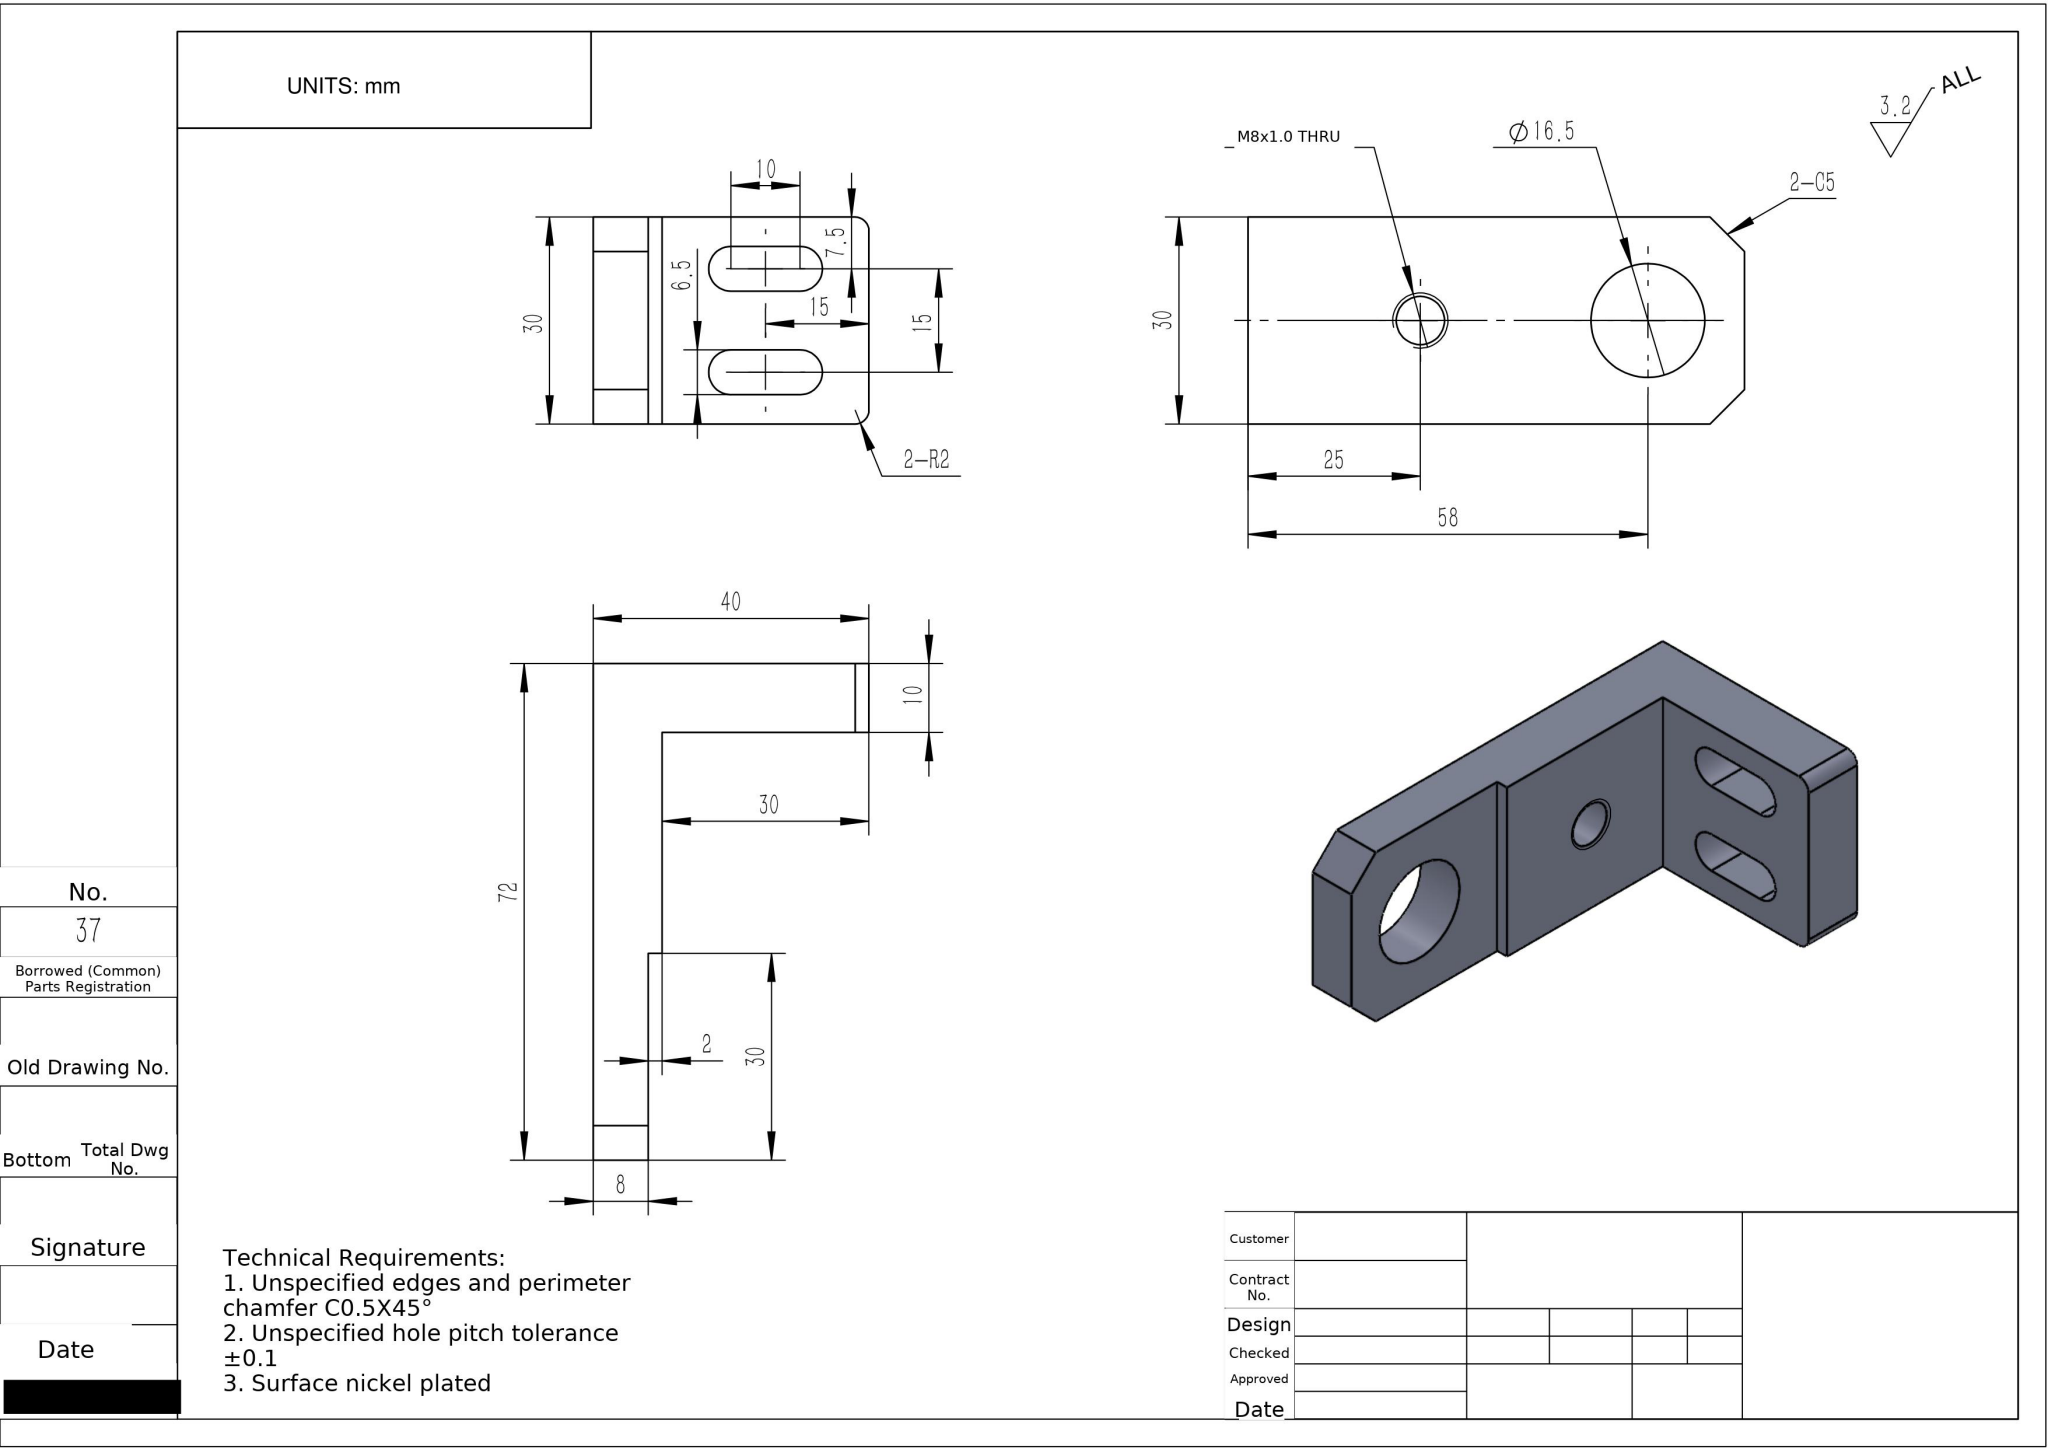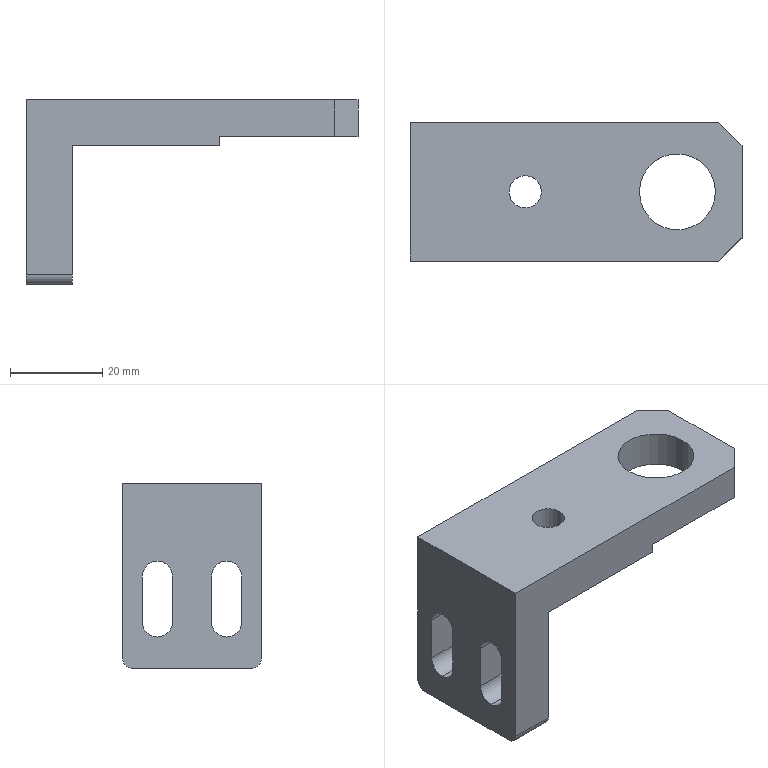Part | NX | mm | 1 solid | 28 faces | box 72 x 30 x 40 mm | volume 24524 mm3 | plane 16 | cylinder 12 | commonest cylinder face diameters 6.5 x6 16.5 x2 7 x2 4 x2
STEP:
#1=COLOUR_RGB('',0.7922,0.8196,0.9333);
#2=FILL_AREA_STYLE_COLOUR('',#1);
#3=FILL_AREA_STYLE('',(#2));
#4=SURFACE_STYLE_FILL_AREA(#3);
#5=SURFACE_SIDE_STYLE('',(#4));
#6=SURFACE_STYLE_USAGE(.BOTH.,#5);
#7=PRESENTATION_STYLE_ASSIGNMENT((#6));
#8=CARTESIAN_POINT('',(30.25,0.,2.));
#9=VERTEX_POINT('',#8);
#10=CARTESIAN_POINT('',(13.75,0.,2.));
#11=VERTEX_POINT('',#10);
#12=CARTESIAN_POINT('',(22.,0.,2.));
#13=DIRECTION('',(0.,0.,-1.));
#14=DIRECTION('',(-1.,0.,0.));
#15=AXIS2_PLACEMENT_3D('',#12,#13,#14);
#16=CIRCLE('',#15,8.25);
#17=EDGE_CURVE('',#9,#11,#16,.T.);
#18=ORIENTED_EDGE('',*,*,#17,.T.);
#19=CARTESIAN_POINT('',(13.75,0.,10.));
#20=VERTEX_POINT('',#19);
#21=CARTESIAN_POINT('',(13.75,0.,10.));
#22=DIRECTION('',(0.,0.,1.));
#23=VECTOR('',#22,1000.);
#24=LINE('',#21,#23);
#25=EDGE_CURVE('',#11,#20,#24,.T.);
#26=ORIENTED_EDGE('',*,*,#25,.T.);
#27=CARTESIAN_POINT('',(30.25,0.,10.));
#28=VERTEX_POINT('',#27);
#29=CARTESIAN_POINT('',(22.,0.,10.));
#30=DIRECTION('',(0.,0.,1.));
#31=DIRECTION('',(1.,0.,0.));
#32=AXIS2_PLACEMENT_3D('',#29,#30,#31);
#33=CIRCLE('',#32,8.25);
#34=EDGE_CURVE('',#20,#28,#33,.T.);
#35=ORIENTED_EDGE('',*,*,#34,.T.);
#36=CARTESIAN_POINT('',(30.25,0.,10.));
#37=DIRECTION('',(0.,0.,1.));
#38=VECTOR('',#37,1000.);
#39=LINE('',#36,#38);
#40=EDGE_CURVE('',#9,#28,#39,.T.);
#41=ORIENTED_EDGE('',*,*,#40,.F.);
#42=EDGE_LOOP('',(#18,#26,#35,#41));
#43=FACE_OUTER_BOUND('',#42,.T.);
#44=CARTESIAN_POINT('',(22.,0.,10.));
#45=DIRECTION('',(0.,0.,1.));
#46=DIRECTION('',(1.,0.,0.));
#47=AXIS2_PLACEMENT_3D('',#44,#45,#46);
#48=CYLINDRICAL_SURFACE('',#47,8.25);
#49=ADVANCED_FACE('',(#43),#48,.F.);
#50=CARTESIAN_POINT('',(-7.5,-0.,10.));
#51=VERTEX_POINT('',#50);
#52=CARTESIAN_POINT('',(-14.5,-0.,10.));
#53=VERTEX_POINT('',#52);
#54=CARTESIAN_POINT('',(-11.,-0.,10.));
#55=DIRECTION('',(0.,0.,-1.));
#56=DIRECTION('',(-1.,0.,0.));
#57=AXIS2_PLACEMENT_3D('',#54,#55,#56);
#58=CIRCLE('',#57,3.5);
#59=EDGE_CURVE('',#51,#53,#58,.T.);
#60=ORIENTED_EDGE('',*,*,#59,.F.);
#61=CARTESIAN_POINT('',(-7.5,-0.,-0.));
#62=VERTEX_POINT('',#61);
#63=CARTESIAN_POINT('',(-7.5,-0.,0.));
#64=DIRECTION('',(0.,0.,-1.));
#65=VECTOR('',#64,1000.);
#66=LINE('',#63,#65);
#67=EDGE_CURVE('',#51,#62,#66,.T.);
#68=ORIENTED_EDGE('',*,*,#67,.T.);
#69=CARTESIAN_POINT('',(-14.5,-0.,-0.));
#70=VERTEX_POINT('',#69);
#71=CARTESIAN_POINT('',(-11.,-0.,-0.));
#72=DIRECTION('',(0.,0.,-1.));
#73=DIRECTION('',(-1.,0.,0.));
#74=AXIS2_PLACEMENT_3D('',#71,#72,#73);
#75=CIRCLE('',#74,3.5);
#76=EDGE_CURVE('',#62,#70,#75,.T.);
#77=ORIENTED_EDGE('',*,*,#76,.T.);
#78=CARTESIAN_POINT('',(-14.5,-0.,0.));
#79=DIRECTION('',(0.,0.,-1.));
#80=VECTOR('',#79,1000.);
#81=LINE('',#78,#80);
#82=EDGE_CURVE('',#53,#70,#81,.T.);
#83=ORIENTED_EDGE('',*,*,#82,.F.);
#84=EDGE_LOOP('',(#60,#68,#77,#83));
#85=FACE_OUTER_BOUND('',#84,.T.);
#86=CARTESIAN_POINT('',(-11.,-0.,0.));
#87=DIRECTION('',(0.,0.,-1.));
#88=DIRECTION('',(-1.,0.,0.));
#89=AXIS2_PLACEMENT_3D('',#86,#87,#88);
#90=CYLINDRICAL_SURFACE('',#89,3.5);
#91=ADVANCED_FACE('',(#85),#90,.F.);
#92=CARTESIAN_POINT('',(-36.,-7.5,-23.25));
#93=VERTEX_POINT('',#92);
#94=CARTESIAN_POINT('',(-36.,-4.25,-20.));
#95=VERTEX_POINT('',#94);
#96=CARTESIAN_POINT('',(-36.,-7.5,-20.));
#97=DIRECTION('',(1.,0.,0.));
#98=DIRECTION('',(0.,0.,1.));
#99=AXIS2_PLACEMENT_3D('',#96,#97,#98);
#100=CIRCLE('',#99,3.25);
#101=EDGE_CURVE('',#93,#95,#100,.T.);
#102=ORIENTED_EDGE('',*,*,#101,.F.);
#103=CARTESIAN_POINT('',(-26.,-7.5,-23.25));
#104=VERTEX_POINT('',#103);
#105=CARTESIAN_POINT('',(-36.,-7.5,-23.25));
#106=DIRECTION('',(1.,0.,0.));
#107=VECTOR('',#106,1000.);
#108=LINE('',#105,#107);
#109=EDGE_CURVE('',#93,#104,#108,.T.);
#110=ORIENTED_EDGE('',*,*,#109,.T.);
#111=CARTESIAN_POINT('',(-26.,-4.25,-20.));
#112=VERTEX_POINT('',#111);
#113=CARTESIAN_POINT('',(-26.,-7.5,-20.));
#114=DIRECTION('',(1.,0.,0.));
#115=DIRECTION('',(0.,0.,1.));
#116=AXIS2_PLACEMENT_3D('',#113,#114,#115);
#117=CIRCLE('',#116,3.25);
#118=EDGE_CURVE('',#104,#112,#117,.T.);
#119=ORIENTED_EDGE('',*,*,#118,.T.);
#120=CARTESIAN_POINT('',(-36.,-4.25,-20.));
#121=DIRECTION('',(1.,0.,0.));
#122=VECTOR('',#121,1000.);
#123=LINE('',#120,#122);
#124=EDGE_CURVE('',#95,#112,#123,.T.);
#125=ORIENTED_EDGE('',*,*,#124,.F.);
#126=EDGE_LOOP('',(#102,#110,#119,#125));
#127=FACE_OUTER_BOUND('',#126,.T.);
#128=CARTESIAN_POINT('',(-36.,-7.5,-20.));
#129=DIRECTION('',(1.,0.,0.));
#130=DIRECTION('',(0.,0.,-1.));
#131=AXIS2_PLACEMENT_3D('',#128,#129,#130);
#132=CYLINDRICAL_SURFACE('',#131,3.25);
#133=ADVANCED_FACE('',(#127),#132,.F.);
#134=CARTESIAN_POINT('',(-36.,7.5,-23.25));
#135=VERTEX_POINT('',#134);
#136=CARTESIAN_POINT('',(-36.,10.75,-20.));
#137=VERTEX_POINT('',#136);
#138=CARTESIAN_POINT('',(-36.,7.5,-20.));
#139=DIRECTION('',(1.,0.,0.));
#140=DIRECTION('',(0.,0.,-1.));
#141=AXIS2_PLACEMENT_3D('',#138,#139,#140);
#142=CIRCLE('',#141,3.25);
#143=EDGE_CURVE('',#135,#137,#142,.T.);
#144=ORIENTED_EDGE('',*,*,#143,.F.);
#145=CARTESIAN_POINT('',(-26.,7.5,-23.25));
#146=VERTEX_POINT('',#145);
#147=CARTESIAN_POINT('',(-36.,7.5,-23.25));
#148=DIRECTION('',(1.,0.,0.));
#149=VECTOR('',#148,1000.);
#150=LINE('',#147,#149);
#151=EDGE_CURVE('',#135,#146,#150,.T.);
#152=ORIENTED_EDGE('',*,*,#151,.T.);
#153=CARTESIAN_POINT('',(-26.,10.75,-20.));
#154=VERTEX_POINT('',#153);
#155=CARTESIAN_POINT('',(-26.,7.5,-20.));
#156=DIRECTION('',(1.,0.,0.));
#157=DIRECTION('',(0.,0.,-1.));
#158=AXIS2_PLACEMENT_3D('',#155,#156,#157);
#159=CIRCLE('',#158,3.25);
#160=EDGE_CURVE('',#146,#154,#159,.T.);
#161=ORIENTED_EDGE('',*,*,#160,.T.);
#162=CARTESIAN_POINT('',(-36.,10.75,-20.));
#163=DIRECTION('',(1.,0.,0.));
#164=VECTOR('',#163,1000.);
#165=LINE('',#162,#164);
#166=EDGE_CURVE('',#137,#154,#165,.T.);
#167=ORIENTED_EDGE('',*,*,#166,.F.);
#168=EDGE_LOOP('',(#144,#152,#161,#167));
#169=FACE_OUTER_BOUND('',#168,.T.);
#170=CARTESIAN_POINT('',(-36.,7.5,-20.));
#171=DIRECTION('',(1.,0.,0.));
#172=DIRECTION('',(0.,0.,-1.));
#173=AXIS2_PLACEMENT_3D('',#170,#171,#172);
#174=CYLINDRICAL_SURFACE('',#173,3.25);
#175=ADVANCED_FACE('',(#169),#174,.F.);
#176=CARTESIAN_POINT('',(-11.,-0.,-0.));
#177=DIRECTION('',(0.,0.,-1.));
#178=DIRECTION('',(-1.,0.,0.));
#179=AXIS2_PLACEMENT_3D('',#176,#177,#178);
#180=CIRCLE('',#179,3.5);
#181=EDGE_CURVE('',#70,#62,#180,.T.);
#182=ORIENTED_EDGE('',*,*,#181,.F.);
#183=ORIENTED_EDGE('',*,*,#76,.F.);
#184=EDGE_LOOP('',(#182,#183));
#185=FACE_BOUND('',#184,.T.);
#186=CARTESIAN_POINT('',(-26.,15.,0.));
#187=VERTEX_POINT('',#186);
#188=CARTESIAN_POINT('',(-26.,-15.,0.));
#189=VERTEX_POINT('',#188);
#190=CARTESIAN_POINT('',(-26.,15.,0.));
#191=DIRECTION('',(0.,-1.,0.));
#192=VECTOR('',#191,1000.);
#193=LINE('',#190,#192);
#194=EDGE_CURVE('',#187,#189,#193,.T.);
#195=ORIENTED_EDGE('',*,*,#194,.F.);
#196=CARTESIAN_POINT('',(6.,15.,0.));
#197=VERTEX_POINT('',#196);
#198=CARTESIAN_POINT('',(-36.,15.,0.));
#199=DIRECTION('',(-1.,0.,0.));
#200=VECTOR('',#199,1000.);
#201=LINE('',#198,#200);
#202=EDGE_CURVE('',#197,#187,#201,.T.);
#203=ORIENTED_EDGE('',*,*,#202,.F.);
#204=CARTESIAN_POINT('',(6.,-15.,0.));
#205=VERTEX_POINT('',#204);
#206=CARTESIAN_POINT('',(6.,15.,0.));
#207=DIRECTION('',(0.,1.,0.));
#208=VECTOR('',#207,1000.);
#209=LINE('',#206,#208);
#210=EDGE_CURVE('',#205,#197,#209,.T.);
#211=ORIENTED_EDGE('',*,*,#210,.F.);
#212=CARTESIAN_POINT('',(-36.,-15.,0.));
#213=DIRECTION('',(1.,0.,0.));
#214=VECTOR('',#213,1000.);
#215=LINE('',#212,#214);
#216=EDGE_CURVE('',#189,#205,#215,.T.);
#217=ORIENTED_EDGE('',*,*,#216,.F.);
#218=EDGE_LOOP('',(#195,#203,#211,#217));
#219=FACE_OUTER_BOUND('',#218,.T.);
#220=CARTESIAN_POINT('',(36.,-15.,0.));
#221=DIRECTION('',(0.,0.,1.));
#222=DIRECTION('',(1.,0.,0.));
#223=AXIS2_PLACEMENT_3D('',#220,#221,#222);
#224=PLANE('',#223);
#225=ADVANCED_FACE('',(#185,#219),#224,.F.);
#226=CARTESIAN_POINT('',(36.,-10.,10.));
#227=VERTEX_POINT('',#226);
#228=CARTESIAN_POINT('',(36.,10.,10.));
#229=VERTEX_POINT('',#228);
#230=CARTESIAN_POINT('',(36.,15.,10.));
#231=DIRECTION('',(-0.,1.,0.));
#232=VECTOR('',#231,1000.);
#233=LINE('',#230,#232);
#234=EDGE_CURVE('',#227,#229,#233,.T.);
#235=ORIENTED_EDGE('',*,*,#234,.F.);
#236=CARTESIAN_POINT('',(36.,-10.,2.));
#237=VERTEX_POINT('',#236);
#238=CARTESIAN_POINT('',(36.,-10.,10.));
#239=DIRECTION('',(0.,0.,-1.));
#240=VECTOR('',#239,1000.);
#241=LINE('',#238,#240);
#242=EDGE_CURVE('',#227,#237,#241,.T.);
#243=ORIENTED_EDGE('',*,*,#242,.T.);
#244=CARTESIAN_POINT('',(36.,10.,2.));
#245=VERTEX_POINT('',#244);
#246=CARTESIAN_POINT('',(36.,15.,2.));
#247=DIRECTION('',(0.,-1.,0.));
#248=VECTOR('',#247,1000.);
#249=LINE('',#246,#248);
#250=EDGE_CURVE('',#245,#237,#249,.T.);
#251=ORIENTED_EDGE('',*,*,#250,.F.);
#252=CARTESIAN_POINT('',(36.,10.,10.));
#253=DIRECTION('',(0.,0.,1.));
#254=VECTOR('',#253,1000.);
#255=LINE('',#252,#254);
#256=EDGE_CURVE('',#245,#229,#255,.T.);
#257=ORIENTED_EDGE('',*,*,#256,.T.);
#258=EDGE_LOOP('',(#235,#243,#251,#257));
#259=FACE_OUTER_BOUND('',#258,.T.);
#260=CARTESIAN_POINT('',(36.,15.,10.));
#261=DIRECTION('',(-1.,-0.,0.));
#262=DIRECTION('',(0.,-1.,0.));
#263=AXIS2_PLACEMENT_3D('',#260,#261,#262);
#264=PLANE('',#263);
#265=ADVANCED_FACE('',(#259),#264,.F.);
#266=CARTESIAN_POINT('',(31.,15.,10.));
#267=VERTEX_POINT('',#266);
#268=CARTESIAN_POINT('',(-36.,15.,10.));
#269=VERTEX_POINT('',#268);
#270=CARTESIAN_POINT('',(-36.,15.,10.));
#271=DIRECTION('',(-1.,0.,0.));
#272=VECTOR('',#271,1000.);
#273=LINE('',#270,#272);
#274=EDGE_CURVE('',#267,#269,#273,.T.);
#275=ORIENTED_EDGE('',*,*,#274,.F.);
#276=CARTESIAN_POINT('',(31.,15.,2.));
#277=VERTEX_POINT('',#276);
#278=CARTESIAN_POINT('',(31.,15.,10.));
#279=DIRECTION('',(0.,0.,-1.));
#280=VECTOR('',#279,1000.);
#281=LINE('',#278,#280);
#282=EDGE_CURVE('',#267,#277,#281,.T.);
#283=ORIENTED_EDGE('',*,*,#282,.T.);
#284=CARTESIAN_POINT('',(6.,15.,2.));
#285=VERTEX_POINT('',#284);
#286=CARTESIAN_POINT('',(36.,15.,2.));
#287=DIRECTION('',(1.,0.,0.));
#288=VECTOR('',#287,1000.);
#289=LINE('',#286,#288);
#290=EDGE_CURVE('',#285,#277,#289,.T.);
#291=ORIENTED_EDGE('',*,*,#290,.F.);
#292=CARTESIAN_POINT('',(6.,15.,2.));
#293=DIRECTION('',(0.,0.,-1.));
#294=VECTOR('',#293,1000.);
#295=LINE('',#292,#294);
#296=EDGE_CURVE('',#285,#197,#295,.T.);
#297=ORIENTED_EDGE('',*,*,#296,.T.);
#298=ORIENTED_EDGE('',*,*,#202,.T.);
#299=CARTESIAN_POINT('',(-26.,15.,-28.));
#300=VERTEX_POINT('',#299);
#301=CARTESIAN_POINT('',(-26.,15.,-30.));
#302=DIRECTION('',(0.,0.,1.));
#303=VECTOR('',#302,1000.);
#304=LINE('',#301,#303);
#305=EDGE_CURVE('',#300,#187,#304,.T.);
#306=ORIENTED_EDGE('',*,*,#305,.F.);
#307=CARTESIAN_POINT('',(-36.,15.,-28.));
#308=VERTEX_POINT('',#307);
#309=CARTESIAN_POINT('',(-36.,15.,-28.));
#310=DIRECTION('',(-1.,0.,0.));
#311=VECTOR('',#310,1000.);
#312=LINE('',#309,#311);
#313=EDGE_CURVE('',#300,#308,#312,.T.);
#314=ORIENTED_EDGE('',*,*,#313,.T.);
#315=CARTESIAN_POINT('',(-36.,15.,10.));
#316=DIRECTION('',(0.,0.,-1.));
#317=VECTOR('',#316,1000.);
#318=LINE('',#315,#317);
#319=EDGE_CURVE('',#269,#308,#318,.T.);
#320=ORIENTED_EDGE('',*,*,#319,.F.);
#321=EDGE_LOOP('',(#275,#283,#291,#297,#298,#306,#314,#320));
#322=FACE_OUTER_BOUND('',#321,.T.);
#323=CARTESIAN_POINT('',(-36.,15.,10.));
#324=DIRECTION('',(0.,-1.,0.));
#325=DIRECTION('',(0.,0.,-1.));
#326=AXIS2_PLACEMENT_3D('',#323,#324,#325);
#327=PLANE('',#326);
#328=ADVANCED_FACE('',(#322),#327,.F.);
#329=CARTESIAN_POINT('',(-36.,-4.25,-10.));
#330=VERTEX_POINT('',#329);
#331=CARTESIAN_POINT('',(-36.,-4.25,-10.));
#332=DIRECTION('',(0.,-0.,1.));
#333=VECTOR('',#332,1000.);
#334=LINE('',#331,#333);
#335=EDGE_CURVE('',#95,#330,#334,.T.);
#336=ORIENTED_EDGE('',*,*,#335,.T.);
#337=CARTESIAN_POINT('',(-36.,-10.75,-10.));
#338=VERTEX_POINT('',#337);
#339=CARTESIAN_POINT('',(-36.,-7.5,-10.));
#340=DIRECTION('',(1.,0.,0.));
#341=DIRECTION('',(0.,0.,1.));
#342=AXIS2_PLACEMENT_3D('',#339,#340,#341);
#343=CIRCLE('',#342,3.25);
#344=EDGE_CURVE('',#330,#338,#343,.T.);
#345=ORIENTED_EDGE('',*,*,#344,.T.);
#346=CARTESIAN_POINT('',(-36.,-10.75,-20.));
#347=VERTEX_POINT('',#346);
#348=CARTESIAN_POINT('',(-36.,-10.75,-10.));
#349=DIRECTION('',(0.,0.,-1.));
#350=VECTOR('',#349,1000.);
#351=LINE('',#348,#350);
#352=EDGE_CURVE('',#338,#347,#351,.T.);
#353=ORIENTED_EDGE('',*,*,#352,.T.);
#354=CARTESIAN_POINT('',(-36.,-7.5,-20.));
#355=DIRECTION('',(1.,0.,0.));
#356=DIRECTION('',(0.,0.,1.));
#357=AXIS2_PLACEMENT_3D('',#354,#355,#356);
#358=CIRCLE('',#357,3.25);
#359=EDGE_CURVE('',#347,#93,#358,.T.);
#360=ORIENTED_EDGE('',*,*,#359,.T.);
#361=ORIENTED_EDGE('',*,*,#101,.T.);
#362=EDGE_LOOP('',(#336,#345,#353,#360,#361));
#363=FACE_BOUND('',#362,.T.);
#364=CARTESIAN_POINT('',(-36.,10.75,-10.));
#365=VERTEX_POINT('',#364);
#366=CARTESIAN_POINT('',(-36.,10.75,-10.));
#367=DIRECTION('',(0.,-0.,1.));
#368=VECTOR('',#367,1000.);
#369=LINE('',#366,#368);
#370=EDGE_CURVE('',#137,#365,#369,.T.);
#371=ORIENTED_EDGE('',*,*,#370,.T.);
#372=CARTESIAN_POINT('',(-36.,4.25,-10.));
#373=VERTEX_POINT('',#372);
#374=CARTESIAN_POINT('',(-36.,7.5,-10.));
#375=DIRECTION('',(1.,0.,0.));
#376=DIRECTION('',(0.,0.,-1.));
#377=AXIS2_PLACEMENT_3D('',#374,#375,#376);
#378=CIRCLE('',#377,3.25);
#379=EDGE_CURVE('',#365,#373,#378,.T.);
#380=ORIENTED_EDGE('',*,*,#379,.T.);
#381=CARTESIAN_POINT('',(-36.,4.25,-20.));
#382=VERTEX_POINT('',#381);
#383=CARTESIAN_POINT('',(-36.,4.25,-10.));
#384=DIRECTION('',(0.,0.,-1.));
#385=VECTOR('',#384,1000.);
#386=LINE('',#383,#385);
#387=EDGE_CURVE('',#373,#382,#386,.T.);
#388=ORIENTED_EDGE('',*,*,#387,.T.);
#389=CARTESIAN_POINT('',(-36.,7.5,-20.));
#390=DIRECTION('',(1.,0.,0.));
#391=DIRECTION('',(0.,0.,-1.));
#392=AXIS2_PLACEMENT_3D('',#389,#390,#391);
#393=CIRCLE('',#392,3.25);
#394=EDGE_CURVE('',#382,#135,#393,.T.);
#395=ORIENTED_EDGE('',*,*,#394,.T.);
#396=ORIENTED_EDGE('',*,*,#143,.T.);
#397=EDGE_LOOP('',(#371,#380,#388,#395,#396));
#398=FACE_BOUND('',#397,.T.);
#399=ORIENTED_EDGE('',*,*,#319,.T.);
#400=CARTESIAN_POINT('',(-36.,13.,-30.));
#401=VERTEX_POINT('',#400);
#402=CARTESIAN_POINT('',(-36.,13.,-28.));
#403=DIRECTION('',(-1.,0.,0.));
#404=DIRECTION('',(0.,1.,0.));
#405=AXIS2_PLACEMENT_3D('',#402,#403,#404);
#406=CIRCLE('',#405,2.);
#407=EDGE_CURVE('',#308,#401,#406,.T.);
#408=ORIENTED_EDGE('',*,*,#407,.T.);
#409=CARTESIAN_POINT('',(-36.,-13.,-30.));
#410=VERTEX_POINT('',#409);
#411=CARTESIAN_POINT('',(-36.,15.,-30.));
#412=DIRECTION('',(0.,1.,0.));
#413=VECTOR('',#412,1000.);
#414=LINE('',#411,#413);
#415=EDGE_CURVE('',#410,#401,#414,.T.);
#416=ORIENTED_EDGE('',*,*,#415,.F.);
#417=CARTESIAN_POINT('',(-36.,-15.,-28.));
#418=VERTEX_POINT('',#417);
#419=CARTESIAN_POINT('',(-36.,-13.,-28.));
#420=DIRECTION('',(-1.,0.,0.));
#421=DIRECTION('',(0.,1.,0.));
#422=AXIS2_PLACEMENT_3D('',#419,#420,#421);
#423=CIRCLE('',#422,2.);
#424=EDGE_CURVE('',#410,#418,#423,.T.);
#425=ORIENTED_EDGE('',*,*,#424,.T.);
#426=CARTESIAN_POINT('',(-36.,-15.,10.));
#427=VERTEX_POINT('',#426);
#428=CARTESIAN_POINT('',(-36.,-15.,10.));
#429=DIRECTION('',(0.,0.,-1.));
#430=VECTOR('',#429,1000.);
#431=LINE('',#428,#430);
#432=EDGE_CURVE('',#427,#418,#431,.T.);
#433=ORIENTED_EDGE('',*,*,#432,.F.);
#434=CARTESIAN_POINT('',(-36.,15.,10.));
#435=DIRECTION('',(-0.,-1.,0.));
#436=VECTOR('',#435,1000.);
#437=LINE('',#434,#436);
#438=EDGE_CURVE('',#269,#427,#437,.T.);
#439=ORIENTED_EDGE('',*,*,#438,.F.);
#440=EDGE_LOOP('',(#399,#408,#416,#425,#433,#439));
#441=FACE_OUTER_BOUND('',#440,.T.);
#442=CARTESIAN_POINT('',(-36.,15.,10.));
#443=DIRECTION('',(1.,-0.,0.));
#444=DIRECTION('',(0.,1.,0.));
#445=AXIS2_PLACEMENT_3D('',#442,#443,#444);
#446=PLANE('',#445);
#447=ADVANCED_FACE('',(#363,#398,#441),#446,.F.);
#448=CARTESIAN_POINT('',(31.,-15.,2.));
#449=VERTEX_POINT('',#448);
#450=CARTESIAN_POINT('',(6.,-15.,2.));
#451=VERTEX_POINT('',#450);
#452=CARTESIAN_POINT('',(36.,-15.,2.));
#453=DIRECTION('',(-1.,0.,0.));
#454=VECTOR('',#453,1000.);
#455=LINE('',#452,#454);
#456=EDGE_CURVE('',#449,#451,#455,.T.);
#457=ORIENTED_EDGE('',*,*,#456,.F.);
#458=CARTESIAN_POINT('',(31.,-15.,10.));
#459=VERTEX_POINT('',#458);
#460=CARTESIAN_POINT('',(31.,-15.,10.));
#461=DIRECTION('',(0.,0.,1.));
#462=VECTOR('',#461,1000.);
#463=LINE('',#460,#462);
#464=EDGE_CURVE('',#449,#459,#463,.T.);
#465=ORIENTED_EDGE('',*,*,#464,.T.);
#466=CARTESIAN_POINT('',(-36.,-15.,10.));
#467=DIRECTION('',(1.,0.,0.));
#468=VECTOR('',#467,1000.);
#469=LINE('',#466,#468);
#470=EDGE_CURVE('',#427,#459,#469,.T.);
#471=ORIENTED_EDGE('',*,*,#470,.F.);
#472=ORIENTED_EDGE('',*,*,#432,.T.);
#473=CARTESIAN_POINT('',(-26.,-15.,-28.));
#474=VERTEX_POINT('',#473);
#475=CARTESIAN_POINT('',(-26.,-15.,-28.));
#476=DIRECTION('',(1.,0.,0.));
#477=VECTOR('',#476,1000.);
#478=LINE('',#475,#477);
#479=EDGE_CURVE('',#418,#474,#478,.T.);
#480=ORIENTED_EDGE('',*,*,#479,.T.);
#481=CARTESIAN_POINT('',(-26.,-15.,-30.));
#482=DIRECTION('',(0.,0.,1.));
#483=VECTOR('',#482,1000.);
#484=LINE('',#481,#483);
#485=EDGE_CURVE('',#474,#189,#484,.T.);
#486=ORIENTED_EDGE('',*,*,#485,.T.);
#487=ORIENTED_EDGE('',*,*,#216,.T.);
#488=CARTESIAN_POINT('',(6.,-15.,2.));
#489=DIRECTION('',(0.,0.,-1.));
#490=VECTOR('',#489,1000.);
#491=LINE('',#488,#490);
#492=EDGE_CURVE('',#451,#205,#491,.T.);
#493=ORIENTED_EDGE('',*,*,#492,.F.);
#494=EDGE_LOOP('',(#457,#465,#471,#472,#480,#486,#487,#493));
#495=FACE_OUTER_BOUND('',#494,.T.);
#496=CARTESIAN_POINT('',(-36.,-15.,10.));
#497=DIRECTION('',(0.,1.,0.));
#498=DIRECTION('',(0.,0.,1.));
#499=AXIS2_PLACEMENT_3D('',#496,#497,#498);
#500=PLANE('',#499);
#501=ADVANCED_FACE('',(#495),#500,.F.);
#502=CARTESIAN_POINT('',(22.,0.,10.));
#503=DIRECTION('',(0.,0.,1.));
#504=DIRECTION('',(1.,0.,0.));
#505=AXIS2_PLACEMENT_3D('',#502,#503,#504);
#506=CIRCLE('',#505,8.25);
#507=EDGE_CURVE('',#28,#20,#506,.T.);
#508=ORIENTED_EDGE('',*,*,#507,.F.);
#509=ORIENTED_EDGE('',*,*,#34,.F.);
#510=EDGE_LOOP('',(#508,#509));
#511=FACE_BOUND('',#510,.T.);
#512=CARTESIAN_POINT('',(-11.,-0.,10.));
#513=DIRECTION('',(0.,0.,-1.));
#514=DIRECTION('',(-1.,0.,0.));
#515=AXIS2_PLACEMENT_3D('',#512,#513,#514);
#516=CIRCLE('',#515,3.5);
#517=EDGE_CURVE('',#53,#51,#516,.T.);
#518=ORIENTED_EDGE('',*,*,#517,.T.);
#519=ORIENTED_EDGE('',*,*,#59,.T.);
#520=EDGE_LOOP('',(#518,#519));
#521=FACE_BOUND('',#520,.T.);
#522=ORIENTED_EDGE('',*,*,#470,.T.);
#523=CARTESIAN_POINT('',(33.5,-12.5,10.));
#524=DIRECTION('',(0.7071,0.7071,0.));
#525=VECTOR('',#524,1000.);
#526=LINE('',#523,#525);
#527=EDGE_CURVE('',#459,#227,#526,.T.);
#528=ORIENTED_EDGE('',*,*,#527,.T.);
#529=ORIENTED_EDGE('',*,*,#234,.T.);
#530=CARTESIAN_POINT('',(48.5,-2.5,10.));
#531=DIRECTION('',(-0.7071,0.7071,0.));
#532=VECTOR('',#531,1000.);
#533=LINE('',#530,#532);
#534=EDGE_CURVE('',#229,#267,#533,.T.);
#535=ORIENTED_EDGE('',*,*,#534,.T.);
#536=ORIENTED_EDGE('',*,*,#274,.T.);
#537=ORIENTED_EDGE('',*,*,#438,.T.);
#538=EDGE_LOOP('',(#522,#528,#529,#535,#536,#537));
#539=FACE_OUTER_BOUND('',#538,.T.);
#540=CARTESIAN_POINT('',(36.,-15.,10.));
#541=DIRECTION('',(0.,0.,1.));
#542=DIRECTION('',(1.,0.,0.));
#543=AXIS2_PLACEMENT_3D('',#540,#541,#542);
#544=PLANE('',#543);
#545=ADVANCED_FACE('',(#511,#521,#539),#544,.T.);
#546=ORIENTED_EDGE('',*,*,#210,.T.);
#547=ORIENTED_EDGE('',*,*,#296,.F.);
#548=CARTESIAN_POINT('',(6.,15.,2.));
#549=DIRECTION('',(0.,1.,0.));
#550=VECTOR('',#549,1000.);
#551=LINE('',#548,#550);
#552=EDGE_CURVE('',#451,#285,#551,.T.);
#553=ORIENTED_EDGE('',*,*,#552,.F.);
#554=ORIENTED_EDGE('',*,*,#492,.T.);
#555=EDGE_LOOP('',(#546,#547,#553,#554));
#556=FACE_OUTER_BOUND('',#555,.T.);
#557=CARTESIAN_POINT('',(6.,15.,2.));
#558=DIRECTION('',(-1.,0.,0.));
#559=DIRECTION('',(-0.,-1.,0.));
#560=AXIS2_PLACEMENT_3D('',#557,#558,#559);
#561=PLANE('',#560);
#562=ADVANCED_FACE('',(#556),#561,.F.);
#563=ORIENTED_EDGE('',*,*,#17,.F.);
#564=CARTESIAN_POINT('',(22.,0.,2.));
#565=DIRECTION('',(0.,0.,-1.));
#566=DIRECTION('',(-1.,0.,0.));
#567=AXIS2_PLACEMENT_3D('',#564,#565,#566);
#568=CIRCLE('',#567,8.25);
#569=EDGE_CURVE('',#11,#9,#568,.T.);
#570=ORIENTED_EDGE('',*,*,#569,.F.);
#571=EDGE_LOOP('',(#563,#570));
#572=FACE_BOUND('',#571,.T.);
#573=ORIENTED_EDGE('',*,*,#250,.T.);
#574=CARTESIAN_POINT('',(33.5,-12.5,2.));
#575=DIRECTION('',(-0.7071,-0.7071,0.));
#576=VECTOR('',#575,1000.);
#577=LINE('',#574,#576);
#578=EDGE_CURVE('',#237,#449,#577,.T.);
#579=ORIENTED_EDGE('',*,*,#578,.T.);
#580=ORIENTED_EDGE('',*,*,#456,.T.);
#581=ORIENTED_EDGE('',*,*,#552,.T.);
#582=ORIENTED_EDGE('',*,*,#290,.T.);
#583=CARTESIAN_POINT('',(48.5,-2.5,2.));
#584=DIRECTION('',(0.7071,-0.7071,0.));
#585=VECTOR('',#584,1000.);
#586=LINE('',#583,#585);
#587=EDGE_CURVE('',#277,#245,#586,.T.);
#588=ORIENTED_EDGE('',*,*,#587,.T.);
#589=EDGE_LOOP('',(#573,#579,#580,#581,#582,#588));
#590=FACE_OUTER_BOUND('',#589,.T.);
#591=CARTESIAN_POINT('',(36.,-15.,2.));
#592=DIRECTION('',(0.,0.,-1.));
#593=DIRECTION('',(-1.,0.,0.));
#594=AXIS2_PLACEMENT_3D('',#591,#592,#593);
#595=PLANE('',#594);
#596=ADVANCED_FACE('',(#572,#590),#595,.T.);
#597=CARTESIAN_POINT('',(-26.,-10.75,-10.));
#598=VERTEX_POINT('',#597);
#599=CARTESIAN_POINT('',(-26.,-10.75,-20.));
#600=VERTEX_POINT('',#599);
#601=CARTESIAN_POINT('',(-26.,-10.75,-10.));
#602=DIRECTION('',(0.,0.,-1.));
#603=VECTOR('',#602,1000.);
#604=LINE('',#601,#603);
#605=EDGE_CURVE('',#598,#600,#604,.T.);
#606=ORIENTED_EDGE('',*,*,#605,.F.);
#607=CARTESIAN_POINT('',(-26.,-4.25,-10.));
#608=VERTEX_POINT('',#607);
#609=CARTESIAN_POINT('',(-26.,-7.5,-10.));
#610=DIRECTION('',(1.,0.,0.));
#611=DIRECTION('',(0.,0.,1.));
#612=AXIS2_PLACEMENT_3D('',#609,#610,#611);
#613=CIRCLE('',#612,3.25);
#614=EDGE_CURVE('',#608,#598,#613,.T.);
#615=ORIENTED_EDGE('',*,*,#614,.F.);
#616=CARTESIAN_POINT('',(-26.,-4.25,-10.));
#617=DIRECTION('',(0.,-0.,1.));
#618=VECTOR('',#617,1000.);
#619=LINE('',#616,#618);
#620=EDGE_CURVE('',#112,#608,#619,.T.);
#621=ORIENTED_EDGE('',*,*,#620,.F.);
#622=ORIENTED_EDGE('',*,*,#118,.F.);
#623=CARTESIAN_POINT('',(-26.,-7.5,-20.));
#624=DIRECTION('',(1.,0.,0.));
#625=DIRECTION('',(0.,0.,1.));
#626=AXIS2_PLACEMENT_3D('',#623,#624,#625);
#627=CIRCLE('',#626,3.25);
#628=EDGE_CURVE('',#600,#104,#627,.T.);
#629=ORIENTED_EDGE('',*,*,#628,.F.);
#630=EDGE_LOOP('',(#606,#615,#621,#622,#629));
#631=FACE_BOUND('',#630,.T.);
#632=CARTESIAN_POINT('',(-26.,4.25,-10.));
#633=VERTEX_POINT('',#632);
#634=CARTESIAN_POINT('',(-26.,4.25,-20.));
#635=VERTEX_POINT('',#634);
#636=CARTESIAN_POINT('',(-26.,4.25,-10.));
#637=DIRECTION('',(0.,0.,-1.));
#638=VECTOR('',#637,1000.);
#639=LINE('',#636,#638);
#640=EDGE_CURVE('',#633,#635,#639,.T.);
#641=ORIENTED_EDGE('',*,*,#640,.F.);
#642=CARTESIAN_POINT('',(-26.,10.75,-10.));
#643=VERTEX_POINT('',#642);
#644=CARTESIAN_POINT('',(-26.,7.5,-10.));
#645=DIRECTION('',(1.,0.,0.));
#646=DIRECTION('',(0.,0.,-1.));
#647=AXIS2_PLACEMENT_3D('',#644,#645,#646);
#648=CIRCLE('',#647,3.25);
#649=EDGE_CURVE('',#643,#633,#648,.T.);
#650=ORIENTED_EDGE('',*,*,#649,.F.);
#651=CARTESIAN_POINT('',(-26.,10.75,-10.));
#652=DIRECTION('',(0.,-0.,1.));
#653=VECTOR('',#652,1000.);
#654=LINE('',#651,#653);
#655=EDGE_CURVE('',#154,#643,#654,.T.);
#656=ORIENTED_EDGE('',*,*,#655,.F.);
#657=ORIENTED_EDGE('',*,*,#160,.F.);
#658=CARTESIAN_POINT('',(-26.,7.5,-20.));
#659=DIRECTION('',(1.,0.,0.));
#660=DIRECTION('',(0.,0.,-1.));
#661=AXIS2_PLACEMENT_3D('',#658,#659,#660);
#662=CIRCLE('',#661,3.25);
#663=EDGE_CURVE('',#635,#146,#662,.T.);
#664=ORIENTED_EDGE('',*,*,#663,.F.);
#665=EDGE_LOOP('',(#641,#650,#656,#657,#664));
#666=FACE_BOUND('',#665,.T.);
#667=CARTESIAN_POINT('',(-26.,13.,-30.));
#668=VERTEX_POINT('',#667);
#669=CARTESIAN_POINT('',(-26.,-13.,-30.));
#670=VERTEX_POINT('',#669);
#671=CARTESIAN_POINT('',(-26.,15.,-30.));
#672=DIRECTION('',(0.,-1.,0.));
#673=VECTOR('',#672,1000.);
#674=LINE('',#671,#673);
#675=EDGE_CURVE('',#668,#670,#674,.T.);
#676=ORIENTED_EDGE('',*,*,#675,.F.);
#677=CARTESIAN_POINT('',(-26.,13.,-28.));
#678=DIRECTION('',(1.,0.,0.));
#679=DIRECTION('',(0.,0.,1.));
#680=AXIS2_PLACEMENT_3D('',#677,#678,#679);
#681=CIRCLE('',#680,2.);
#682=EDGE_CURVE('',#668,#300,#681,.T.);
#683=ORIENTED_EDGE('',*,*,#682,.T.);
#684=ORIENTED_EDGE('',*,*,#305,.T.);
#685=ORIENTED_EDGE('',*,*,#194,.T.);
#686=ORIENTED_EDGE('',*,*,#485,.F.);
#687=CARTESIAN_POINT('',(-26.,-13.,-28.));
#688=DIRECTION('',(1.,0.,0.));
#689=DIRECTION('',(0.,0.,1.));
#690=AXIS2_PLACEMENT_3D('',#687,#688,#689);
#691=CIRCLE('',#690,2.);
#692=EDGE_CURVE('',#474,#670,#691,.T.);
#693=ORIENTED_EDGE('',*,*,#692,.T.);
#694=EDGE_LOOP('',(#676,#683,#684,#685,#686,#693));
#695=FACE_OUTER_BOUND('',#694,.T.);
#696=CARTESIAN_POINT('',(-26.,15.,-30.));
#697=DIRECTION('',(-1.,0.,0.));
#698=DIRECTION('',(0.,0.,1.));
#699=AXIS2_PLACEMENT_3D('',#696,#697,#698);
#700=PLANE('',#699);
#701=ADVANCED_FACE('',(#631,#666,#695),#700,.F.);
#702=ORIENTED_EDGE('',*,*,#415,.T.);
#703=CARTESIAN_POINT('',(-26.,13.,-30.));
#704=DIRECTION('',(1.,0.,0.));
#705=VECTOR('',#704,1000.);
#706=LINE('',#703,#705);
#707=EDGE_CURVE('',#401,#668,#706,.T.);
#708=ORIENTED_EDGE('',*,*,#707,.T.);
#709=ORIENTED_EDGE('',*,*,#675,.T.);
#710=CARTESIAN_POINT('',(-36.,-13.,-30.));
#711=DIRECTION('',(-1.,0.,0.));
#712=VECTOR('',#711,1000.);
#713=LINE('',#710,#712);
#714=EDGE_CURVE('',#670,#410,#713,.T.);
#715=ORIENTED_EDGE('',*,*,#714,.T.);
#716=EDGE_LOOP('',(#702,#708,#709,#715));
#717=FACE_OUTER_BOUND('',#716,.T.);
#718=CARTESIAN_POINT('',(-26.,-15.,-30.));
#719=DIRECTION('',(0.,0.,-1.));
#720=DIRECTION('',(-1.,0.,0.));
#721=AXIS2_PLACEMENT_3D('',#718,#719,#720);
#722=PLANE('',#721);
#723=ADVANCED_FACE('',(#717),#722,.T.);
#724=ORIENTED_EDGE('',*,*,#649,.T.);
#725=CARTESIAN_POINT('',(-36.,4.25,-10.));
#726=DIRECTION('',(1.,0.,0.));
#727=VECTOR('',#726,1000.);
#728=LINE('',#725,#727);
#729=EDGE_CURVE('',#373,#633,#728,.T.);
#730=ORIENTED_EDGE('',*,*,#729,.F.);
#731=ORIENTED_EDGE('',*,*,#379,.F.);
#732=CARTESIAN_POINT('',(-36.,10.75,-10.));
#733=DIRECTION('',(1.,0.,0.));
#734=VECTOR('',#733,1000.);
#735=LINE('',#732,#734);
#736=EDGE_CURVE('',#365,#643,#735,.T.);
#737=ORIENTED_EDGE('',*,*,#736,.T.);
#738=EDGE_LOOP('',(#724,#730,#731,#737));
#739=FACE_OUTER_BOUND('',#738,.T.);
#740=CARTESIAN_POINT('',(-36.,7.5,-10.));
#741=DIRECTION('',(1.,0.,0.));
#742=DIRECTION('',(0.,0.,-1.));
#743=AXIS2_PLACEMENT_3D('',#740,#741,#742);
#744=CYLINDRICAL_SURFACE('',#743,3.25);
#745=ADVANCED_FACE('',(#739),#744,.F.);
#746=ORIENTED_EDGE('',*,*,#655,.T.);
#747=ORIENTED_EDGE('',*,*,#736,.F.);
#748=ORIENTED_EDGE('',*,*,#370,.F.);
#749=ORIENTED_EDGE('',*,*,#166,.T.);
#750=EDGE_LOOP('',(#746,#747,#748,#749));
#751=FACE_OUTER_BOUND('',#750,.T.);
#752=CARTESIAN_POINT('',(-36.,10.75,-10.));
#753=DIRECTION('',(0.,1.,0.));
#754=DIRECTION('',(0.,-0.,1.));
#755=AXIS2_PLACEMENT_3D('',#752,#753,#754);
#756=PLANE('',#755);
#757=ADVANCED_FACE('',(#751),#756,.F.);
#758=ORIENTED_EDGE('',*,*,#151,.F.);
#759=ORIENTED_EDGE('',*,*,#394,.F.);
#760=CARTESIAN_POINT('',(-36.,4.25,-20.));
#761=DIRECTION('',(1.,0.,0.));
#762=VECTOR('',#761,1000.);
#763=LINE('',#760,#762);
#764=EDGE_CURVE('',#382,#635,#763,.T.);
#765=ORIENTED_EDGE('',*,*,#764,.T.);
#766=ORIENTED_EDGE('',*,*,#663,.T.);
#767=EDGE_LOOP('',(#758,#759,#765,#766));
#768=FACE_OUTER_BOUND('',#767,.T.);
#769=CARTESIAN_POINT('',(-36.,7.5,-20.));
#770=DIRECTION('',(1.,0.,0.));
#771=DIRECTION('',(0.,0.,-1.));
#772=AXIS2_PLACEMENT_3D('',#769,#770,#771);
#773=CYLINDRICAL_SURFACE('',#772,3.25);
#774=ADVANCED_FACE('',(#768),#773,.F.);
#775=ORIENTED_EDGE('',*,*,#640,.T.);
#776=ORIENTED_EDGE('',*,*,#764,.F.);
#777=ORIENTED_EDGE('',*,*,#387,.F.);
#778=ORIENTED_EDGE('',*,*,#729,.T.);
#779=EDGE_LOOP('',(#775,#776,#777,#778));
#780=FACE_OUTER_BOUND('',#779,.T.);
#781=CARTESIAN_POINT('',(-36.,4.25,-10.));
#782=DIRECTION('',(0.,-1.,-0.));
#783=DIRECTION('',(0.,0.,-1.));
#784=AXIS2_PLACEMENT_3D('',#781,#782,#783);
#785=PLANE('',#784);
#786=ADVANCED_FACE('',(#780),#785,.F.);
#787=ORIENTED_EDGE('',*,*,#614,.T.);
#788=CARTESIAN_POINT('',(-36.,-10.75,-10.));
#789=DIRECTION('',(1.,0.,0.));
#790=VECTOR('',#789,1000.);
#791=LINE('',#788,#790);
#792=EDGE_CURVE('',#338,#598,#791,.T.);
#793=ORIENTED_EDGE('',*,*,#792,.F.);
#794=ORIENTED_EDGE('',*,*,#344,.F.);
#795=CARTESIAN_POINT('',(-36.,-4.25,-10.));
#796=DIRECTION('',(1.,0.,0.));
#797=VECTOR('',#796,1000.);
#798=LINE('',#795,#797);
#799=EDGE_CURVE('',#330,#608,#798,.T.);
#800=ORIENTED_EDGE('',*,*,#799,.T.);
#801=EDGE_LOOP('',(#787,#793,#794,#800));
#802=FACE_OUTER_BOUND('',#801,.T.);
#803=CARTESIAN_POINT('',(-36.,-7.5,-10.));
#804=DIRECTION('',(1.,0.,0.));
#805=DIRECTION('',(0.,0.,-1.));
#806=AXIS2_PLACEMENT_3D('',#803,#804,#805);
#807=CYLINDRICAL_SURFACE('',#806,3.25);
#808=ADVANCED_FACE('',(#802),#807,.F.);
#809=ORIENTED_EDGE('',*,*,#620,.T.);
#810=ORIENTED_EDGE('',*,*,#799,.F.);
#811=ORIENTED_EDGE('',*,*,#335,.F.);
#812=ORIENTED_EDGE('',*,*,#124,.T.);
#813=EDGE_LOOP('',(#809,#810,#811,#812));
#814=FACE_OUTER_BOUND('',#813,.T.);
#815=CARTESIAN_POINT('',(-36.,-4.25,-10.));
#816=DIRECTION('',(0.,1.,0.));
#817=DIRECTION('',(0.,-0.,1.));
#818=AXIS2_PLACEMENT_3D('',#815,#816,#817);
#819=PLANE('',#818);
#820=ADVANCED_FACE('',(#814),#819,.F.);
#821=ORIENTED_EDGE('',*,*,#109,.F.);
#822=ORIENTED_EDGE('',*,*,#359,.F.);
#823=CARTESIAN_POINT('',(-36.,-10.75,-20.));
#824=DIRECTION('',(1.,0.,0.));
#825=VECTOR('',#824,1000.);
#826=LINE('',#823,#825);
#827=EDGE_CURVE('',#347,#600,#826,.T.);
#828=ORIENTED_EDGE('',*,*,#827,.T.);
#829=ORIENTED_EDGE('',*,*,#628,.T.);
#830=EDGE_LOOP('',(#821,#822,#828,#829));
#831=FACE_OUTER_BOUND('',#830,.T.);
#832=CARTESIAN_POINT('',(-36.,-7.5,-20.));
#833=DIRECTION('',(1.,0.,0.));
#834=DIRECTION('',(0.,0.,-1.));
#835=AXIS2_PLACEMENT_3D('',#832,#833,#834);
#836=CYLINDRICAL_SURFACE('',#835,3.25);
#837=ADVANCED_FACE('',(#831),#836,.F.);
#838=ORIENTED_EDGE('',*,*,#605,.T.);
#839=ORIENTED_EDGE('',*,*,#827,.F.);
#840=ORIENTED_EDGE('',*,*,#352,.F.);
#841=ORIENTED_EDGE('',*,*,#792,.T.);
#842=EDGE_LOOP('',(#838,#839,#840,#841));
#843=FACE_OUTER_BOUND('',#842,.T.);
#844=CARTESIAN_POINT('',(-36.,-10.75,-10.));
#845=DIRECTION('',(0.,-1.,-0.));
#846=DIRECTION('',(0.,0.,-1.));
#847=AXIS2_PLACEMENT_3D('',#844,#845,#846);
#848=PLANE('',#847);
#849=ADVANCED_FACE('',(#843),#848,.F.);
#850=ORIENTED_EDGE('',*,*,#407,.F.);
#851=ORIENTED_EDGE('',*,*,#313,.F.);
#852=ORIENTED_EDGE('',*,*,#682,.F.);
#853=ORIENTED_EDGE('',*,*,#707,.F.);
#854=EDGE_LOOP('',(#850,#851,#852,#853));
#855=FACE_OUTER_BOUND('',#854,.T.);
#856=CARTESIAN_POINT('',(-26.,13.,-28.));
#857=DIRECTION('',(-1.,0.,0.));
#858=DIRECTION('',(0.,0.,1.));
#859=AXIS2_PLACEMENT_3D('',#856,#857,#858);
#860=CYLINDRICAL_SURFACE('',#859,2.);
#861=ADVANCED_FACE('',(#855),#860,.T.);
#862=ORIENTED_EDGE('',*,*,#692,.F.);
#863=ORIENTED_EDGE('',*,*,#479,.F.);
#864=ORIENTED_EDGE('',*,*,#424,.F.);
#865=ORIENTED_EDGE('',*,*,#714,.F.);
#866=EDGE_LOOP('',(#862,#863,#864,#865));
#867=FACE_OUTER_BOUND('',#866,.T.);
#868=CARTESIAN_POINT('',(-26.,-13.,-28.));
#869=DIRECTION('',(1.,0.,0.));
#870=DIRECTION('',(0.,0.,-1.));
#871=AXIS2_PLACEMENT_3D('',#868,#869,#870);
#872=CYLINDRICAL_SURFACE('',#871,2.);
#873=ADVANCED_FACE('',(#867),#872,.T.);
#874=ORIENTED_EDGE('',*,*,#527,.F.);
#875=ORIENTED_EDGE('',*,*,#464,.F.);
#876=ORIENTED_EDGE('',*,*,#578,.F.);
#877=ORIENTED_EDGE('',*,*,#242,.F.);
#878=EDGE_LOOP('',(#874,#875,#876,#877));
#879=FACE_OUTER_BOUND('',#878,.T.);
#880=CARTESIAN_POINT('',(36.,-10.,10.));
#881=DIRECTION('',(-0.7071,0.7071,0.));
#882=DIRECTION('',(-0.7071,-0.7071,0.));
#883=AXIS2_PLACEMENT_3D('',#880,#881,#882);
#884=PLANE('',#883);
#885=ADVANCED_FACE('',(#879),#884,.F.);
#886=ORIENTED_EDGE('',*,*,#534,.F.);
#887=ORIENTED_EDGE('',*,*,#256,.F.);
#888=ORIENTED_EDGE('',*,*,#587,.F.);
#889=ORIENTED_EDGE('',*,*,#282,.F.);
#890=EDGE_LOOP('',(#886,#887,#888,#889));
#891=FACE_OUTER_BOUND('',#890,.T.);
#892=CARTESIAN_POINT('',(31.,15.,10.));
#893=DIRECTION('',(-0.7071,-0.7071,0.));
#894=DIRECTION('',(0.7071,-0.7071,0.));
#895=AXIS2_PLACEMENT_3D('',#892,#893,#894);
#896=PLANE('',#895);
#897=ADVANCED_FACE('',(#891),#896,.F.);
#898=ORIENTED_EDGE('',*,*,#67,.F.);
#899=ORIENTED_EDGE('',*,*,#517,.F.);
#900=ORIENTED_EDGE('',*,*,#82,.T.);
#901=ORIENTED_EDGE('',*,*,#181,.T.);
#902=EDGE_LOOP('',(#898,#899,#900,#901));
#903=FACE_OUTER_BOUND('',#902,.T.);
#904=CARTESIAN_POINT('',(-11.,-0.,0.));
#905=DIRECTION('',(0.,0.,-1.));
#906=DIRECTION('',(-1.,0.,0.));
#907=AXIS2_PLACEMENT_3D('',#904,#905,#906);
#908=CYLINDRICAL_SURFACE('',#907,3.5);
#909=ADVANCED_FACE('',(#903),#908,.F.);
#910=ORIENTED_EDGE('',*,*,#25,.F.);
#911=ORIENTED_EDGE('',*,*,#569,.T.);
#912=ORIENTED_EDGE('',*,*,#40,.T.);
#913=ORIENTED_EDGE('',*,*,#507,.T.);
#914=EDGE_LOOP('',(#910,#911,#912,#913));
#915=FACE_OUTER_BOUND('',#914,.T.);
#916=CARTESIAN_POINT('',(22.,0.,10.));
#917=DIRECTION('',(0.,0.,1.));
#918=DIRECTION('',(1.,0.,0.));
#919=AXIS2_PLACEMENT_3D('',#916,#917,#918);
#920=CYLINDRICAL_SURFACE('',#919,8.25);
#921=ADVANCED_FACE('',(#915),#920,.F.);
#922=CLOSED_SHELL('',(#49,#91,#133,#175,#225,#265,#328,#447,#501,#545,#562,#596,#701,#723,#745,#757,#774,#786,#808,#820,#837,#849,#861,#873,#885,#897,#909,#921));
#923=MANIFOLD_SOLID_BREP('',#922);
#924=STYLED_ITEM('',(#7),#923);
#925=(LENGTH_UNIT()NAMED_UNIT(*)SI_UNIT(.MILLI.,.METRE.));
#926=UNCERTAINTY_MEASURE_WITH_UNIT(LENGTH_MEASURE(0.00001),#925,'','');
#927=(NAMED_UNIT(*)PLANE_ANGLE_UNIT()SI_UNIT($,.RADIAN.));
#928=(NAMED_UNIT(*)SI_UNIT($,.STERADIAN.)SOLID_ANGLE_UNIT());
#929=(GEOMETRIC_REPRESENTATION_CONTEXT(3)GLOBAL_UNCERTAINTY_ASSIGNED_CONTEXT((#926))GLOBAL_UNIT_ASSIGNED_CONTEXT((#925,#927,#928))REPRESENTATION_CONTEXT('',''));
#930=MECHANICAL_DESIGN_GEOMETRIC_PRESENTATION_REPRESENTATION('',(#924),#929);
#931=PRESENTATION_LAYER_ASSIGNMENT('','',(#924));
#932=CARTESIAN_POINT('',(0.,0.,0.));
#933=DIRECTION('',(0.,0.,1.));
#934=DIRECTION('',(1.,0.,0.));
#935=AXIS2_PLACEMENT_3D('',#932,#933,#934);
#936=(LENGTH_UNIT()NAMED_UNIT(*)SI_UNIT(.MILLI.,.METRE.));
#937=UNCERTAINTY_MEASURE_WITH_UNIT(LENGTH_MEASURE(0.00001),#936,'','');
#938=(NAMED_UNIT(*)PLANE_ANGLE_UNIT()SI_UNIT($,.RADIAN.));
#939=(NAMED_UNIT(*)SI_UNIT($,.STERADIAN.)SOLID_ANGLE_UNIT());
#940=(GEOMETRIC_REPRESENTATION_CONTEXT(3)GLOBAL_UNCERTAINTY_ASSIGNED_CONTEXT((#937))GLOBAL_UNIT_ASSIGNED_CONTEXT((#936,#938,#939))REPRESENTATION_CONTEXT('',''));
#941=ADVANCED_BREP_SHAPE_REPRESENTATION('',(#923,#935),#940);